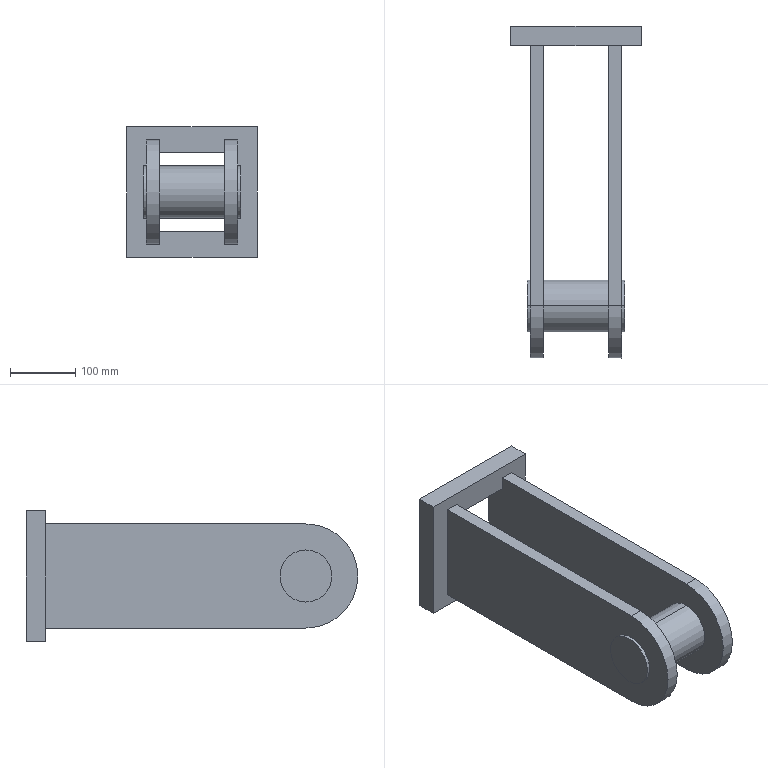Component | SolidWorks | LiftingAndOperatingMechanism-1_20-1 | 1 solid | 26 faces | box 200 x 510 x 200 mm | volume 4355044 mm3 | plane 18 | cylinder 8 | commonest cylinder face diameters 80 x6 160 x2
build123d program:
from build123d import *

# Parameters (mm, degrees)
SKETCH1_W           = 200
SKETCH1_H           = 200
BOSS_EXTRUDE1_DEPTH = 30
BOSS_EXTRUDE2_START = 50
BOSS_EXTRUDE2_DEPTH = 20
SKETCH4_R           = 40
BOSS_EXTRUDE3_DEPTH = 75
SKETCH5_W           = 120
SKETCH5_H           = 100
CUT_EXTRUDE2_DEPTH  = 501.4


with BuildPart() as part:
    # Sketch1 → Boss-Extrude1 (new body)
    with BuildSketch(Plane(origin=(0, 0, 0), x_dir=(1, 0, 0), z_dir=(0, 1, 0))):
        Rectangle(SKETCH1_W, SKETCH1_H)
    extrude(amount=BOSS_EXTRUDE1_DEPTH)

    # Sketch2 → Boss-Extrude2 (add)
    with BuildSketch(Plane.XY.offset(BOSS_EXTRUDE2_START)):
        with BuildLine():
            Line((-80, 430), (-80, 30))
            Line((-80, 30), (80, 30))
            Line((80, 30), (80, 430))
            ThreePointArc((80, 430), (0, 510), (-80, 430))
        make_face()
    boss_extrude2 = extrude(amount=BOSS_EXTRUDE2_DEPTH)

    # Mirror1: Boss-Extrude2 across plane
    add(boss_extrude2.mirror(Plane.XY))

    # Sketch4 → Boss-Extrude3 (add, symmetric)
    with BuildSketch(Plane.XY):
        with Locations(Location((0, 430, 0), (0, 0, 180))):
            Circle(SKETCH4_R)
    extrude(amount=BOSS_EXTRUDE3_DEPTH, both=True)

    # Sketch5 → Cut-Extrude2 (cut, through all)
    with BuildSketch(Plane(origin=(0, 30, 0), x_dir=(1, 0, 0), z_dir=(0, 1, 0))):
        Rectangle(SKETCH5_W, SKETCH5_H)
    extrude(amount=-CUT_EXTRUDE2_DEPTH, mode=Mode.SUBTRACT)


solid = part.part

# Placed as in the assembly
solid = solid.moved(Location((-1438.963, 12438.918, 6252.153), (180, 90, 0)))
STEP:
#1=COLOUR_RGB('',0.7922,0.8196,0.9333);
#2=FILL_AREA_STYLE_COLOUR('',#1);
#3=FILL_AREA_STYLE('',(#2));
#4=SURFACE_STYLE_FILL_AREA(#3);
#5=SURFACE_SIDE_STYLE('',(#4));
#6=SURFACE_STYLE_USAGE(.BOTH.,#5);
#7=PRESENTATION_STYLE_ASSIGNMENT((#6));
#8=CARTESIAN_POINT('',(-59.605,472.792,244.573));
#9=VERTEX_POINT('',#8);
#10=CARTESIAN_POINT('',(-59.605,472.792,247.723));
#11=VERTEX_POINT('',#10);
#12=CARTESIAN_POINT('',(-59.605,472.792,246.148));
#13=DIRECTION('',(-1.,-0.,0.0000002));
#14=DIRECTION('',(-0.0000002,0.,-1.));
#15=AXIS2_PLACEMENT_3D('',#12,#13,#14);
#16=CIRCLE('',#15,1.575);
#17=EDGE_CURVE('',#9,#11,#16,.T.);
#18=ORIENTED_EDGE('',*,*,#17,.F.);
#19=CARTESIAN_POINT('',(-59.408,472.792,244.573));
#20=VERTEX_POINT('',#19);
#21=CARTESIAN_POINT('',(-59.605,472.792,244.573));
#22=DIRECTION('',(1.,0.,-0.0000002));
#23=VECTOR('',#22,39.37);
#24=LINE('',#21,#23);
#25=EDGE_CURVE('',#9,#20,#24,.T.);
#26=ORIENTED_EDGE('',*,*,#25,.T.);
#27=CARTESIAN_POINT('',(-59.408,472.792,247.723));
#28=VERTEX_POINT('',#27);
#29=CARTESIAN_POINT('',(-59.408,472.792,246.148));
#30=DIRECTION('',(1.,0.,-0.0000002));
#31=DIRECTION('',(-0.0000002,0.,-1.));
#32=AXIS2_PLACEMENT_3D('',#29,#30,#31);
#33=CIRCLE('',#32,1.575);
#34=EDGE_CURVE('',#28,#20,#33,.T.);
#35=ORIENTED_EDGE('',*,*,#34,.F.);
#36=CARTESIAN_POINT('',(-59.605,472.792,247.723));
#37=DIRECTION('',(1.,0.,-0.0000002));
#38=VECTOR('',#37,39.37);
#39=LINE('',#36,#38);
#40=EDGE_CURVE('',#11,#28,#39,.T.);
#41=ORIENTED_EDGE('',*,*,#40,.F.);
#42=EDGE_LOOP('',(#18,#26,#35,#41));
#43=FACE_OUTER_BOUND('',#42,.T.);
#44=CARTESIAN_POINT('',(-59.605,472.792,246.148));
#45=DIRECTION('',(1.,0.,-0.0000002));
#46=DIRECTION('',(0.0000002,0.,1.));
#47=AXIS2_PLACEMENT_3D('',#44,#45,#46);
#48=CYLINDRICAL_SURFACE('',#47,1.575);
#49=ADVANCED_FACE('',(#43),#48,.T.);
#50=CARTESIAN_POINT('',(-53.896,472.792,244.573));
#51=VERTEX_POINT('',#50);
#52=CARTESIAN_POINT('',(-53.896,472.792,247.723));
#53=VERTEX_POINT('',#52);
#54=CARTESIAN_POINT('',(-53.896,472.792,246.148));
#55=DIRECTION('',(-1.,-0.,0.0000002));
#56=DIRECTION('',(0.0000002,0.,1.));
#57=AXIS2_PLACEMENT_3D('',#54,#55,#56);
#58=CIRCLE('',#57,1.575);
#59=EDGE_CURVE('',#51,#53,#58,.T.);
#60=ORIENTED_EDGE('',*,*,#59,.F.);
#61=CARTESIAN_POINT('',(-53.699,472.792,244.573));
#62=VERTEX_POINT('',#61);
#63=CARTESIAN_POINT('',(-59.605,472.792,244.573));
#64=DIRECTION('',(1.,0.,-0.0000002));
#65=VECTOR('',#64,39.37);
#66=LINE('',#63,#65);
#67=EDGE_CURVE('',#51,#62,#66,.T.);
#68=ORIENTED_EDGE('',*,*,#67,.T.);
#69=CARTESIAN_POINT('',(-53.699,472.792,247.723));
#70=VERTEX_POINT('',#69);
#71=CARTESIAN_POINT('',(-53.699,472.792,246.148));
#72=DIRECTION('',(-1.,-0.,0.0000002));
#73=DIRECTION('',(-0.0000002,0.,-1.));
#74=AXIS2_PLACEMENT_3D('',#71,#72,#73);
#75=CIRCLE('',#74,1.575);
#76=EDGE_CURVE('',#62,#70,#75,.T.);
#77=ORIENTED_EDGE('',*,*,#76,.T.);
#78=CARTESIAN_POINT('',(-59.605,472.792,247.723));
#79=DIRECTION('',(1.,0.,-0.0000002));
#80=VECTOR('',#79,39.37);
#81=LINE('',#78,#80);
#82=EDGE_CURVE('',#53,#70,#81,.T.);
#83=ORIENTED_EDGE('',*,*,#82,.F.);
#84=EDGE_LOOP('',(#60,#68,#77,#83));
#85=FACE_OUTER_BOUND('',#84,.T.);
#86=CARTESIAN_POINT('',(-59.605,472.792,246.148));
#87=DIRECTION('',(1.,0.,-0.0000002));
#88=DIRECTION('',(0.0000002,0.,1.));
#89=AXIS2_PLACEMENT_3D('',#86,#87,#88);
#90=CYLINDRICAL_SURFACE('',#89,1.575);
#91=ADVANCED_FACE('',(#85),#90,.T.);
#92=CARTESIAN_POINT('',(-58.621,472.792,247.723));
#93=VERTEX_POINT('',#92);
#94=CARTESIAN_POINT('',(-58.621,472.792,244.573));
#95=VERTEX_POINT('',#94);
#96=CARTESIAN_POINT('',(-58.621,472.792,246.148));
#97=DIRECTION('',(1.,0.,-0.0000002));
#98=DIRECTION('',(-0.0000002,0.,-1.));
#99=AXIS2_PLACEMENT_3D('',#96,#97,#98);
#100=CIRCLE('',#99,1.575);
#101=EDGE_CURVE('',#93,#95,#100,.T.);
#102=ORIENTED_EDGE('',*,*,#101,.T.);
#103=CARTESIAN_POINT('',(-54.684,472.792,244.573));
#104=VERTEX_POINT('',#103);
#105=CARTESIAN_POINT('',(-59.605,472.792,244.573));
#106=DIRECTION('',(1.,0.,-0.0000002));
#107=VECTOR('',#106,39.37);
#108=LINE('',#105,#107);
#109=EDGE_CURVE('',#95,#104,#108,.T.);
#110=ORIENTED_EDGE('',*,*,#109,.T.);
#111=CARTESIAN_POINT('',(-54.684,472.792,247.723));
#112=VERTEX_POINT('',#111);
#113=CARTESIAN_POINT('',(-54.684,472.792,246.148));
#114=DIRECTION('',(-1.,-0.,0.0000002));
#115=DIRECTION('',(0.0000002,0.,1.));
#116=AXIS2_PLACEMENT_3D('',#113,#114,#115);
#117=CIRCLE('',#116,1.575);
#118=EDGE_CURVE('',#104,#112,#117,.T.);
#119=ORIENTED_EDGE('',*,*,#118,.T.);
#120=CARTESIAN_POINT('',(-59.605,472.792,247.723));
#121=DIRECTION('',(1.,0.,-0.0000002));
#122=VECTOR('',#121,39.37);
#123=LINE('',#120,#122);
#124=EDGE_CURVE('',#93,#112,#123,.T.);
#125=ORIENTED_EDGE('',*,*,#124,.F.);
#126=EDGE_LOOP('',(#102,#110,#119,#125));
#127=FACE_OUTER_BOUND('',#126,.T.);
#128=CARTESIAN_POINT('',(-59.605,472.792,246.148));
#129=DIRECTION('',(1.,0.,-0.0000002));
#130=DIRECTION('',(0.0000002,0.,1.));
#131=AXIS2_PLACEMENT_3D('',#128,#129,#130);
#132=CYLINDRICAL_SURFACE('',#131,1.575);
#133=ADVANCED_FACE('',(#127),#132,.T.);
#134=CARTESIAN_POINT('',(-60.589,489.721,242.211));
#135=VERTEX_POINT('',#134);
#136=CARTESIAN_POINT('',(-52.715,489.721,242.211));
#137=VERTEX_POINT('',#136);
#138=CARTESIAN_POINT('',(-52.715,489.721,242.211));
#139=DIRECTION('',(1.,0.,-0.0000002));
#140=VECTOR('',#139,39.37);
#141=LINE('',#138,#140);
#142=EDGE_CURVE('',#135,#137,#141,.T.);
#143=ORIENTED_EDGE('',*,*,#142,.T.);
#144=CARTESIAN_POINT('',(-52.715,488.54,242.211));
#145=VERTEX_POINT('',#144);
#146=CARTESIAN_POINT('',(-52.715,488.54,242.211));
#147=DIRECTION('',(-0.,1.,0.));
#148=VECTOR('',#147,39.37);
#149=LINE('',#146,#148);
#150=EDGE_CURVE('',#145,#137,#149,.T.);
#151=ORIENTED_EDGE('',*,*,#150,.F.);
#152=CARTESIAN_POINT('',(-60.589,488.54,242.211));
#153=VERTEX_POINT('',#152);
#154=CARTESIAN_POINT('',(-52.715,488.54,242.211));
#155=DIRECTION('',(1.,0.,-0.0000002));
#156=VECTOR('',#155,39.37);
#157=LINE('',#154,#156);
#158=EDGE_CURVE('',#153,#145,#157,.T.);
#159=ORIENTED_EDGE('',*,*,#158,.F.);
#160=CARTESIAN_POINT('',(-60.589,488.54,242.211));
#161=DIRECTION('',(-0.,1.,0.));
#162=VECTOR('',#161,39.37);
#163=LINE('',#160,#162);
#164=EDGE_CURVE('',#153,#135,#163,.T.);
#165=ORIENTED_EDGE('',*,*,#164,.T.);
#166=EDGE_LOOP('',(#143,#151,#159,#165));
#167=FACE_OUTER_BOUND('',#166,.T.);
#168=CARTESIAN_POINT('',(-52.715,488.54,242.211));
#169=DIRECTION('',(0.0000002,-0.,1.));
#170=DIRECTION('',(-1.,-0.,0.0000002));
#171=AXIS2_PLACEMENT_3D('',#168,#169,#170);
#172=PLANE('',#171);
#173=ADVANCED_FACE('',(#167),#172,.F.);
#174=CARTESIAN_POINT('',(-52.715,489.721,250.085));
#175=VERTEX_POINT('',#174);
#176=CARTESIAN_POINT('',(-52.715,489.721,250.085));
#177=DIRECTION('',(0.0000002,-0.,1.));
#178=VECTOR('',#177,39.37);
#179=LINE('',#176,#178);
#180=EDGE_CURVE('',#137,#175,#179,.T.);
#181=ORIENTED_EDGE('',*,*,#180,.T.);
#182=CARTESIAN_POINT('',(-52.715,488.54,250.085));
#183=VERTEX_POINT('',#182);
#184=CARTESIAN_POINT('',(-52.715,488.54,250.085));
#185=DIRECTION('',(-0.,1.,0.));
#186=VECTOR('',#185,39.37);
#187=LINE('',#184,#186);
#188=EDGE_CURVE('',#183,#175,#187,.T.);
#189=ORIENTED_EDGE('',*,*,#188,.F.);
#190=CARTESIAN_POINT('',(-52.715,488.54,250.085));
#191=DIRECTION('',(0.0000002,-0.,1.));
#192=VECTOR('',#191,39.37);
#193=LINE('',#190,#192);
#194=EDGE_CURVE('',#145,#183,#193,.T.);
#195=ORIENTED_EDGE('',*,*,#194,.F.);
#196=ORIENTED_EDGE('',*,*,#150,.T.);
#197=EDGE_LOOP('',(#181,#189,#195,#196));
#198=FACE_OUTER_BOUND('',#197,.T.);
#199=CARTESIAN_POINT('',(-52.715,488.54,250.085));
#200=DIRECTION('',(-1.,-0.,0.0000002));
#201=DIRECTION('',(-0.0000002,0.,-1.));
#202=AXIS2_PLACEMENT_3D('',#199,#200,#201);
#203=PLANE('',#202);
#204=ADVANCED_FACE('',(#198),#203,.F.);
#205=CARTESIAN_POINT('',(-60.589,489.721,250.085));
#206=VERTEX_POINT('',#205);
#207=CARTESIAN_POINT('',(-52.715,489.721,250.085));
#208=DIRECTION('',(-1.,-0.,0.0000002));
#209=VECTOR('',#208,39.37);
#210=LINE('',#207,#209);
#211=EDGE_CURVE('',#175,#206,#210,.T.);
#212=ORIENTED_EDGE('',*,*,#211,.T.);
#213=CARTESIAN_POINT('',(-60.589,488.54,250.085));
#214=VERTEX_POINT('',#213);
#215=CARTESIAN_POINT('',(-60.589,488.54,250.085));
#216=DIRECTION('',(-0.,1.,0.));
#217=VECTOR('',#216,39.37);
#218=LINE('',#215,#217);
#219=EDGE_CURVE('',#214,#206,#218,.T.);
#220=ORIENTED_EDGE('',*,*,#219,.F.);
#221=CARTESIAN_POINT('',(-52.715,488.54,250.085));
#222=DIRECTION('',(-1.,-0.,0.0000002));
#223=VECTOR('',#222,39.37);
#224=LINE('',#221,#223);
#225=EDGE_CURVE('',#183,#214,#224,.T.);
#226=ORIENTED_EDGE('',*,*,#225,.F.);
#227=ORIENTED_EDGE('',*,*,#188,.T.);
#228=EDGE_LOOP('',(#212,#220,#226,#227));
#229=FACE_OUTER_BOUND('',#228,.T.);
#230=CARTESIAN_POINT('',(-52.715,488.54,250.085));
#231=DIRECTION('',(-0.0000002,0.,-1.));
#232=DIRECTION('',(1.,0.,-0.0000002));
#233=AXIS2_PLACEMENT_3D('',#230,#231,#232);
#234=PLANE('',#233);
#235=ADVANCED_FACE('',(#229),#234,.F.);
#236=CARTESIAN_POINT('',(-60.589,489.721,250.085));
#237=DIRECTION('',(-0.0000002,0.,-1.));
#238=VECTOR('',#237,39.37);
#239=LINE('',#236,#238);
#240=EDGE_CURVE('',#206,#135,#239,.T.);
#241=ORIENTED_EDGE('',*,*,#240,.T.);
#242=ORIENTED_EDGE('',*,*,#164,.F.);
#243=CARTESIAN_POINT('',(-60.589,488.54,250.085));
#244=DIRECTION('',(-0.0000002,0.,-1.));
#245=VECTOR('',#244,39.37);
#246=LINE('',#243,#245);
#247=EDGE_CURVE('',#214,#153,#246,.T.);
#248=ORIENTED_EDGE('',*,*,#247,.F.);
#249=ORIENTED_EDGE('',*,*,#219,.T.);
#250=EDGE_LOOP('',(#241,#242,#248,#249));
#251=FACE_OUTER_BOUND('',#250,.T.);
#252=CARTESIAN_POINT('',(-60.589,488.54,250.085));
#253=DIRECTION('',(1.,0.,-0.0000002));
#254=DIRECTION('',(0.0000002,-0.,1.));
#255=AXIS2_PLACEMENT_3D('',#252,#253,#254);
#256=PLANE('',#255);
#257=ADVANCED_FACE('',(#251),#256,.F.);
#258=CARTESIAN_POINT('',(-58.621,488.54,243.786));
#259=VERTEX_POINT('',#258);
#260=CARTESIAN_POINT('',(-54.684,488.54,243.786));
#261=VERTEX_POINT('',#260);
#262=CARTESIAN_POINT('',(-54.684,488.54,243.786));
#263=DIRECTION('',(1.,0.,-0.0000002));
#264=VECTOR('',#263,39.37);
#265=LINE('',#262,#264);
#266=EDGE_CURVE('',#259,#261,#265,.T.);
#267=ORIENTED_EDGE('',*,*,#266,.F.);
#268=CARTESIAN_POINT('',(-58.621,488.54,242.998));
#269=VERTEX_POINT('',#268);
#270=CARTESIAN_POINT('',(-58.621,488.54,246.148));
#271=DIRECTION('',(-0.0000002,-0.,-1.));
#272=VECTOR('',#271,39.37);
#273=LINE('',#270,#272);
#274=EDGE_CURVE('',#259,#269,#273,.T.);
#275=ORIENTED_EDGE('',*,*,#274,.T.);
#276=CARTESIAN_POINT('',(-59.408,488.54,242.998));
#277=VERTEX_POINT('',#276);
#278=CARTESIAN_POINT('',(-59.408,488.54,242.998));
#279=DIRECTION('',(1.,0.,-0.0000002));
#280=VECTOR('',#279,39.37);
#281=LINE('',#278,#280);
#282=EDGE_CURVE('',#277,#269,#281,.T.);
#283=ORIENTED_EDGE('',*,*,#282,.F.);
#284=CARTESIAN_POINT('',(-59.408,488.54,249.297));
#285=VERTEX_POINT('',#284);
#286=CARTESIAN_POINT('',(-59.408,488.54,246.148));
#287=DIRECTION('',(-0.0000002,-0.,-1.));
#288=VECTOR('',#287,39.37);
#289=LINE('',#286,#288);
#290=EDGE_CURVE('',#285,#277,#289,.T.);
#291=ORIENTED_EDGE('',*,*,#290,.F.);
#292=CARTESIAN_POINT('',(-58.621,488.54,249.297));
#293=VERTEX_POINT('',#292);
#294=CARTESIAN_POINT('',(-59.408,488.54,249.297));
#295=DIRECTION('',(1.,0.,-0.0000002));
#296=VECTOR('',#295,39.37);
#297=LINE('',#294,#296);
#298=EDGE_CURVE('',#285,#293,#297,.T.);
#299=ORIENTED_EDGE('',*,*,#298,.T.);
#300=CARTESIAN_POINT('',(-58.621,488.54,248.51));
#301=VERTEX_POINT('',#300);
#302=CARTESIAN_POINT('',(-58.621,488.54,246.148));
#303=DIRECTION('',(-0.0000002,-0.,-1.));
#304=VECTOR('',#303,39.37);
#305=LINE('',#302,#304);
#306=EDGE_CURVE('',#293,#301,#305,.T.);
#307=ORIENTED_EDGE('',*,*,#306,.T.);
#308=CARTESIAN_POINT('',(-54.684,488.54,248.51));
#309=VERTEX_POINT('',#308);
#310=CARTESIAN_POINT('',(-54.684,488.54,248.51));
#311=DIRECTION('',(-1.,-0.,0.0000002));
#312=VECTOR('',#311,39.37);
#313=LINE('',#310,#312);
#314=EDGE_CURVE('',#309,#301,#313,.T.);
#315=ORIENTED_EDGE('',*,*,#314,.F.);
#316=CARTESIAN_POINT('',(-54.684,488.54,249.297));
#317=VERTEX_POINT('',#316);
#318=CARTESIAN_POINT('',(-54.684,488.54,246.148));
#319=DIRECTION('',(-0.0000002,-0.,-1.));
#320=VECTOR('',#319,39.37);
#321=LINE('',#318,#320);
#322=EDGE_CURVE('',#317,#309,#321,.T.);
#323=ORIENTED_EDGE('',*,*,#322,.F.);
#324=CARTESIAN_POINT('',(-53.896,488.54,249.297));
#325=VERTEX_POINT('',#324);
#326=CARTESIAN_POINT('',(-53.896,488.54,249.297));
#327=DIRECTION('',(-1.,-0.,0.0000002));
#328=VECTOR('',#327,39.37);
#329=LINE('',#326,#328);
#330=EDGE_CURVE('',#325,#317,#329,.T.);
#331=ORIENTED_EDGE('',*,*,#330,.F.);
#332=CARTESIAN_POINT('',(-53.896,488.54,242.998));
#333=VERTEX_POINT('',#332);
#334=CARTESIAN_POINT('',(-53.896,488.54,246.148));
#335=DIRECTION('',(-0.0000002,-0.,-1.));
#336=VECTOR('',#335,39.37);
#337=LINE('',#334,#336);
#338=EDGE_CURVE('',#325,#333,#337,.T.);
#339=ORIENTED_EDGE('',*,*,#338,.T.);
#340=CARTESIAN_POINT('',(-54.684,488.54,242.998));
#341=VERTEX_POINT('',#340);
#342=CARTESIAN_POINT('',(-53.896,488.54,242.998));
#343=DIRECTION('',(-1.,-0.,0.0000002));
#344=VECTOR('',#343,39.37);
#345=LINE('',#342,#344);
#346=EDGE_CURVE('',#333,#341,#345,.T.);
#347=ORIENTED_EDGE('',*,*,#346,.T.);
#348=CARTESIAN_POINT('',(-54.684,488.54,246.148));
#349=DIRECTION('',(-0.0000002,-0.,-1.));
#350=VECTOR('',#349,39.37);
#351=LINE('',#348,#350);
#352=EDGE_CURVE('',#261,#341,#351,.T.);
#353=ORIENTED_EDGE('',*,*,#352,.F.);
#354=EDGE_LOOP('',(#267,#275,#283,#291,#299,#307,#315,#323,#331,#339,#347,#353));
#355=FACE_BOUND('',#354,.T.);
#356=ORIENTED_EDGE('',*,*,#158,.T.);
#357=ORIENTED_EDGE('',*,*,#194,.T.);
#358=ORIENTED_EDGE('',*,*,#225,.T.);
#359=ORIENTED_EDGE('',*,*,#247,.T.);
#360=EDGE_LOOP('',(#356,#357,#358,#359));
#361=FACE_OUTER_BOUND('',#360,.T.);
#362=CARTESIAN_POINT('',(-56.652,488.54,246.148));
#363=DIRECTION('',(0.,-1.,-0.));
#364=DIRECTION('',(-1.,-0.,0.0000002));
#365=AXIS2_PLACEMENT_3D('',#362,#363,#364);
#366=PLANE('',#365);
#367=ADVANCED_FACE('',(#355,#361),#366,.T.);
#368=CARTESIAN_POINT('',(-58.621,489.721,248.51));
#369=VERTEX_POINT('',#368);
#370=CARTESIAN_POINT('',(-58.621,489.721,243.786));
#371=VERTEX_POINT('',#370);
#372=CARTESIAN_POINT('',(-58.621,489.721,248.51));
#373=DIRECTION('',(-0.0000002,0.,-1.));
#374=VECTOR('',#373,39.37);
#375=LINE('',#372,#374);
#376=EDGE_CURVE('',#369,#371,#375,.T.);
#377=ORIENTED_EDGE('',*,*,#376,.T.);
#378=CARTESIAN_POINT('',(-54.684,489.721,243.786));
#379=VERTEX_POINT('',#378);
#380=CARTESIAN_POINT('',(-54.684,489.721,243.786));
#381=DIRECTION('',(1.,0.,-0.0000002));
#382=VECTOR('',#381,39.37);
#383=LINE('',#380,#382);
#384=EDGE_CURVE('',#371,#379,#383,.T.);
#385=ORIENTED_EDGE('',*,*,#384,.T.);
#386=CARTESIAN_POINT('',(-54.684,489.721,248.51));
#387=VERTEX_POINT('',#386);
#388=CARTESIAN_POINT('',(-54.684,489.721,248.51));
#389=DIRECTION('',(0.0000002,-0.,1.));
#390=VECTOR('',#389,39.37);
#391=LINE('',#388,#390);
#392=EDGE_CURVE('',#379,#387,#391,.T.);
#393=ORIENTED_EDGE('',*,*,#392,.T.);
#394=CARTESIAN_POINT('',(-54.684,489.721,248.51));
#395=DIRECTION('',(-1.,-0.,0.0000002));
#396=VECTOR('',#395,39.37);
#397=LINE('',#394,#396);
#398=EDGE_CURVE('',#387,#369,#397,.T.);
#399=ORIENTED_EDGE('',*,*,#398,.T.);
#400=EDGE_LOOP('',(#377,#385,#393,#399));
#401=FACE_BOUND('',#400,.T.);
#402=ORIENTED_EDGE('',*,*,#142,.F.);
#403=ORIENTED_EDGE('',*,*,#240,.F.);
#404=ORIENTED_EDGE('',*,*,#211,.F.);
#405=ORIENTED_EDGE('',*,*,#180,.F.);
#406=EDGE_LOOP('',(#402,#403,#404,#405));
#407=FACE_OUTER_BOUND('',#406,.T.);
#408=CARTESIAN_POINT('',(-56.652,489.721,246.148));
#409=DIRECTION('',(0.,-1.,-0.));
#410=DIRECTION('',(-1.,-0.,0.0000002));
#411=AXIS2_PLACEMENT_3D('',#408,#409,#410);
#412=PLANE('',#411);
#413=ADVANCED_FACE('',(#401,#407),#412,.F.);
#414=CARTESIAN_POINT('',(-58.621,472.792,242.998));
#415=VERTEX_POINT('',#414);
#416=CARTESIAN_POINT('',(-58.621,489.721,242.998));
#417=DIRECTION('',(0.,-1.,-0.));
#418=VECTOR('',#417,39.37);
#419=LINE('',#416,#418);
#420=EDGE_CURVE('',#269,#415,#419,.T.);
#421=ORIENTED_EDGE('',*,*,#420,.T.);
#422=CARTESIAN_POINT('',(-59.408,472.792,242.998));
#423=VERTEX_POINT('',#422);
#424=CARTESIAN_POINT('',(-59.408,472.792,242.998));
#425=DIRECTION('',(1.,0.,-0.0000002));
#426=VECTOR('',#425,39.37);
#427=LINE('',#424,#426);
#428=EDGE_CURVE('',#423,#415,#427,.T.);
#429=ORIENTED_EDGE('',*,*,#428,.F.);
#430=CARTESIAN_POINT('',(-59.408,489.721,242.998));
#431=DIRECTION('',(0.,-1.,-0.));
#432=VECTOR('',#431,39.37);
#433=LINE('',#430,#432);
#434=EDGE_CURVE('',#277,#423,#433,.T.);
#435=ORIENTED_EDGE('',*,*,#434,.F.);
#436=ORIENTED_EDGE('',*,*,#282,.T.);
#437=EDGE_LOOP('',(#421,#429,#435,#436));
#438=FACE_OUTER_BOUND('',#437,.T.);
#439=CARTESIAN_POINT('',(-59.408,489.721,242.998));
#440=DIRECTION('',(0.0000002,-0.,1.));
#441=DIRECTION('',(-1.,-0.,0.0000002));
#442=AXIS2_PLACEMENT_3D('',#439,#440,#441);
#443=PLANE('',#442);
#444=ADVANCED_FACE('',(#438),#443,.F.);
#445=CARTESIAN_POINT('',(-58.621,472.792,249.297));
#446=VERTEX_POINT('',#445);
#447=CARTESIAN_POINT('',(-58.621,472.792,246.148));
#448=DIRECTION('',(-1.,-0.,0.0000002));
#449=DIRECTION('',(-0.0000002,0.,-1.));
#450=AXIS2_PLACEMENT_3D('',#447,#448,#449);
#451=CIRCLE('',#450,3.15);
#452=EDGE_CURVE('',#415,#446,#451,.T.);
#453=ORIENTED_EDGE('',*,*,#452,.T.);
#454=CARTESIAN_POINT('',(-59.408,472.792,249.297));
#455=VERTEX_POINT('',#454);
#456=CARTESIAN_POINT('',(-59.408,472.792,249.297));
#457=DIRECTION('',(1.,0.,-0.0000002));
#458=VECTOR('',#457,39.37);
#459=LINE('',#456,#458);
#460=EDGE_CURVE('',#455,#446,#459,.T.);
#461=ORIENTED_EDGE('',*,*,#460,.F.);
#462=CARTESIAN_POINT('',(-59.408,472.792,246.148));
#463=DIRECTION('',(-1.,-0.,0.0000002));
#464=DIRECTION('',(-0.0000002,0.,-1.));
#465=AXIS2_PLACEMENT_3D('',#462,#463,#464);
#466=CIRCLE('',#465,3.15);
#467=EDGE_CURVE('',#423,#455,#466,.T.);
#468=ORIENTED_EDGE('',*,*,#467,.F.);
#469=ORIENTED_EDGE('',*,*,#428,.T.);
#470=EDGE_LOOP('',(#453,#461,#468,#469));
#471=FACE_OUTER_BOUND('',#470,.T.);
#472=CARTESIAN_POINT('',(-59.408,472.792,246.148));
#473=DIRECTION('',(1.,0.,-0.0000002));
#474=DIRECTION('',(0.0000002,0.,1.));
#475=AXIS2_PLACEMENT_3D('',#472,#473,#474);
#476=CYLINDRICAL_SURFACE('',#475,3.15);
#477=ADVANCED_FACE('',(#471),#476,.T.);
#478=CARTESIAN_POINT('',(-58.621,489.721,249.297));
#479=DIRECTION('',(0.,-1.,-0.));
#480=VECTOR('',#479,39.37);
#481=LINE('',#478,#480);
#482=EDGE_CURVE('',#293,#446,#481,.T.);
#483=ORIENTED_EDGE('',*,*,#482,.F.);
#484=ORIENTED_EDGE('',*,*,#298,.F.);
#485=CARTESIAN_POINT('',(-59.408,489.721,249.297));
#486=DIRECTION('',(0.,-1.,-0.));
#487=VECTOR('',#486,39.37);
#488=LINE('',#485,#487);
#489=EDGE_CURVE('',#285,#455,#488,.T.);
#490=ORIENTED_EDGE('',*,*,#489,.T.);
#491=ORIENTED_EDGE('',*,*,#460,.T.);
#492=EDGE_LOOP('',(#483,#484,#490,#491));
#493=FACE_OUTER_BOUND('',#492,.T.);
#494=CARTESIAN_POINT('',(-59.408,489.721,249.297));
#495=DIRECTION('',(0.0000002,-0.,1.));
#496=DIRECTION('',(-1.,-0.,0.0000002));
#497=AXIS2_PLACEMENT_3D('',#494,#495,#496);
#498=PLANE('',#497);
#499=ADVANCED_FACE('',(#493),#498,.T.);
#500=ORIENTED_EDGE('',*,*,#34,.T.);
#501=CARTESIAN_POINT('',(-59.408,472.792,246.148));
#502=DIRECTION('',(1.,0.,-0.0000002));
#503=DIRECTION('',(-0.0000002,0.,-1.));
#504=AXIS2_PLACEMENT_3D('',#501,#502,#503);
#505=CIRCLE('',#504,1.575);
#506=EDGE_CURVE('',#20,#28,#505,.T.);
#507=ORIENTED_EDGE('',*,*,#506,.T.);
#508=EDGE_LOOP('',(#500,#507));
#509=FACE_BOUND('',#508,.T.);
#510=ORIENTED_EDGE('',*,*,#434,.T.);
#511=ORIENTED_EDGE('',*,*,#467,.T.);
#512=ORIENTED_EDGE('',*,*,#489,.F.);
#513=ORIENTED_EDGE('',*,*,#290,.T.);
#514=EDGE_LOOP('',(#510,#511,#512,#513));
#515=FACE_OUTER_BOUND('',#514,.T.);
#516=CARTESIAN_POINT('',(-59.408,489.721,246.148));
#517=DIRECTION('',(-1.,-0.,0.0000002));
#518=DIRECTION('',(-0.0000002,0.,-1.));
#519=AXIS2_PLACEMENT_3D('',#516,#517,#518);
#520=PLANE('',#519);
#521=ADVANCED_FACE('',(#509,#515),#520,.T.);
#522=ORIENTED_EDGE('',*,*,#101,.F.);
#523=CARTESIAN_POINT('',(-58.621,472.792,246.148));
#524=DIRECTION('',(1.,0.,-0.0000002));
#525=DIRECTION('',(-0.0000002,0.,-1.));
#526=AXIS2_PLACEMENT_3D('',#523,#524,#525);
#527=CIRCLE('',#526,1.575);
#528=EDGE_CURVE('',#95,#93,#527,.T.);
#529=ORIENTED_EDGE('',*,*,#528,.F.);
#530=EDGE_LOOP('',(#522,#529));
#531=FACE_BOUND('',#530,.T.);
#532=ORIENTED_EDGE('',*,*,#420,.F.);
#533=ORIENTED_EDGE('',*,*,#274,.F.);
#534=CARTESIAN_POINT('',(-58.621,489.721,243.786));
#535=DIRECTION('',(0.,-1.,-0.));
#536=VECTOR('',#535,39.37);
#537=LINE('',#534,#536);
#538=EDGE_CURVE('',#371,#259,#537,.T.);
#539=ORIENTED_EDGE('',*,*,#538,.F.);
#540=ORIENTED_EDGE('',*,*,#376,.F.);
#541=CARTESIAN_POINT('',(-58.621,489.721,248.51));
#542=DIRECTION('',(0.,-1.,-0.));
#543=VECTOR('',#542,39.37);
#544=LINE('',#541,#543);
#545=EDGE_CURVE('',#369,#301,#544,.T.);
#546=ORIENTED_EDGE('',*,*,#545,.T.);
#547=ORIENTED_EDGE('',*,*,#306,.F.);
#548=ORIENTED_EDGE('',*,*,#482,.T.);
#549=ORIENTED_EDGE('',*,*,#452,.F.);
#550=EDGE_LOOP('',(#532,#533,#539,#540,#546,#547,#548,#549));
#551=FACE_OUTER_BOUND('',#550,.T.);
#552=CARTESIAN_POINT('',(-58.621,489.721,246.148));
#553=DIRECTION('',(-1.,-0.,0.0000002));
#554=DIRECTION('',(-0.0000002,0.,-1.));
#555=AXIS2_PLACEMENT_3D('',#552,#553,#554);
#556=PLANE('',#555);
#557=ADVANCED_FACE('',(#531,#551),#556,.F.);
#558=CARTESIAN_POINT('',(-54.684,472.792,242.998));
#559=VERTEX_POINT('',#558);
#560=CARTESIAN_POINT('',(-54.684,489.721,242.998));
#561=DIRECTION('',(0.,-1.,-0.));
#562=VECTOR('',#561,39.37);
#563=LINE('',#560,#562);
#564=EDGE_CURVE('',#341,#559,#563,.T.);
#565=ORIENTED_EDGE('',*,*,#564,.F.);
#566=ORIENTED_EDGE('',*,*,#346,.F.);
#567=CARTESIAN_POINT('',(-53.896,472.792,242.998));
#568=VERTEX_POINT('',#567);
#569=CARTESIAN_POINT('',(-53.896,489.721,242.998));
#570=DIRECTION('',(0.,-1.,-0.));
#571=VECTOR('',#570,39.37);
#572=LINE('',#569,#571);
#573=EDGE_CURVE('',#333,#568,#572,.T.);
#574=ORIENTED_EDGE('',*,*,#573,.T.);
#575=CARTESIAN_POINT('',(-53.896,472.792,242.998));
#576=DIRECTION('',(-1.,-0.,0.0000002));
#577=VECTOR('',#576,39.37);
#578=LINE('',#575,#577);
#579=EDGE_CURVE('',#568,#559,#578,.T.);
#580=ORIENTED_EDGE('',*,*,#579,.T.);
#581=EDGE_LOOP('',(#565,#566,#574,#580));
#582=FACE_OUTER_BOUND('',#581,.T.);
#583=CARTESIAN_POINT('',(-53.896,489.721,242.998));
#584=DIRECTION('',(-0.0000002,0.,-1.));
#585=DIRECTION('',(1.,0.,-0.0000002));
#586=AXIS2_PLACEMENT_3D('',#583,#584,#585);
#587=PLANE('',#586);
#588=ADVANCED_FACE('',(#582),#587,.T.);
#589=CARTESIAN_POINT('',(-54.684,472.792,249.297));
#590=VERTEX_POINT('',#589);
#591=CARTESIAN_POINT('',(-54.684,489.721,249.297));
#592=DIRECTION('',(0.,-1.,-0.));
#593=VECTOR('',#592,39.37);
#594=LINE('',#591,#593);
#595=EDGE_CURVE('',#317,#590,#594,.T.);
#596=ORIENTED_EDGE('',*,*,#595,.T.);
#597=CARTESIAN_POINT('',(-53.896,472.792,249.297));
#598=VERTEX_POINT('',#597);
#599=CARTESIAN_POINT('',(-53.896,472.792,249.297));
#600=DIRECTION('',(-1.,-0.,0.0000002));
#601=VECTOR('',#600,39.37);
#602=LINE('',#599,#601);
#603=EDGE_CURVE('',#598,#590,#602,.T.);
#604=ORIENTED_EDGE('',*,*,#603,.F.);
#605=CARTESIAN_POINT('',(-53.896,489.721,249.297));
#606=DIRECTION('',(0.,-1.,-0.));
#607=VECTOR('',#606,39.37);
#608=LINE('',#605,#607);
#609=EDGE_CURVE('',#325,#598,#608,.T.);
#610=ORIENTED_EDGE('',*,*,#609,.F.);
#611=ORIENTED_EDGE('',*,*,#330,.T.);
#612=EDGE_LOOP('',(#596,#604,#610,#611));
#613=FACE_OUTER_BOUND('',#612,.T.);
#614=CARTESIAN_POINT('',(-53.896,489.721,249.297));
#615=DIRECTION('',(-0.0000002,0.,-1.));
#616=DIRECTION('',(1.,0.,-0.0000002));
#617=AXIS2_PLACEMENT_3D('',#614,#615,#616);
#618=PLANE('',#617);
#619=ADVANCED_FACE('',(#613),#618,.F.);
#620=CARTESIAN_POINT('',(-54.684,472.792,246.148));
#621=DIRECTION('',(-1.,-0.,0.0000002));
#622=DIRECTION('',(-0.0000002,0.,-1.));
#623=AXIS2_PLACEMENT_3D('',#620,#621,#622);
#624=CIRCLE('',#623,3.15);
#625=EDGE_CURVE('',#559,#590,#624,.T.);
#626=ORIENTED_EDGE('',*,*,#625,.F.);
#627=ORIENTED_EDGE('',*,*,#579,.F.);
#628=CARTESIAN_POINT('',(-53.896,472.792,246.148));
#629=DIRECTION('',(-1.,-0.,0.0000002));
#630=DIRECTION('',(-0.0000002,0.,-1.));
#631=AXIS2_PLACEMENT_3D('',#628,#629,#630);
#632=CIRCLE('',#631,3.15);
#633=EDGE_CURVE('',#568,#598,#632,.T.);
#634=ORIENTED_EDGE('',*,*,#633,.T.);
#635=ORIENTED_EDGE('',*,*,#603,.T.);
#636=EDGE_LOOP('',(#626,#627,#634,#635));
#637=FACE_OUTER_BOUND('',#636,.T.);
#638=CARTESIAN_POINT('',(-53.896,472.792,246.148));
#639=DIRECTION('',(-1.,-0.,0.0000002));
#640=DIRECTION('',(-0.0000002,0.,-1.));
#641=AXIS2_PLACEMENT_3D('',#638,#639,#640);
#642=CYLINDRICAL_SURFACE('',#641,3.15);
#643=ADVANCED_FACE('',(#637),#642,.T.);
#644=CARTESIAN_POINT('',(-53.896,472.792,246.148));
#645=DIRECTION('',(-1.,-0.,0.0000002));
#646=DIRECTION('',(0.0000002,0.,1.));
#647=AXIS2_PLACEMENT_3D('',#644,#645,#646);
#648=CIRCLE('',#647,1.575);
#649=EDGE_CURVE('',#53,#51,#648,.T.);
#650=ORIENTED_EDGE('',*,*,#649,.T.);
#651=ORIENTED_EDGE('',*,*,#59,.T.);
#652=EDGE_LOOP('',(#650,#651));
#653=FACE_BOUND('',#652,.T.);
#654=ORIENTED_EDGE('',*,*,#573,.F.);
#655=ORIENTED_EDGE('',*,*,#338,.F.);
#656=ORIENTED_EDGE('',*,*,#609,.T.);
#657=ORIENTED_EDGE('',*,*,#633,.F.);
#658=EDGE_LOOP('',(#654,#655,#656,#657));
#659=FACE_OUTER_BOUND('',#658,.T.);
#660=CARTESIAN_POINT('',(-53.896,489.721,246.148));
#661=DIRECTION('',(1.,0.,-0.0000002));
#662=DIRECTION('',(-0.0000002,0.,-1.));
#663=AXIS2_PLACEMENT_3D('',#660,#661,#662);
#664=PLANE('',#663);
#665=ADVANCED_FACE('',(#653,#659),#664,.T.);
#666=CARTESIAN_POINT('',(-54.684,472.792,246.148));
#667=DIRECTION('',(-1.,-0.,0.0000002));
#668=DIRECTION('',(0.0000002,0.,1.));
#669=AXIS2_PLACEMENT_3D('',#666,#667,#668);
#670=CIRCLE('',#669,1.575);
#671=EDGE_CURVE('',#112,#104,#670,.T.);
#672=ORIENTED_EDGE('',*,*,#671,.F.);
#673=ORIENTED_EDGE('',*,*,#118,.F.);
#674=EDGE_LOOP('',(#672,#673));
#675=FACE_BOUND('',#674,.T.);
#676=ORIENTED_EDGE('',*,*,#564,.T.);
#677=ORIENTED_EDGE('',*,*,#625,.T.);
#678=ORIENTED_EDGE('',*,*,#595,.F.);
#679=ORIENTED_EDGE('',*,*,#322,.T.);
#680=CARTESIAN_POINT('',(-54.684,489.721,248.51));
#681=DIRECTION('',(0.,-1.,-0.));
#682=VECTOR('',#681,39.37);
#683=LINE('',#680,#682);
#684=EDGE_CURVE('',#387,#309,#683,.T.);
#685=ORIENTED_EDGE('',*,*,#684,.F.);
#686=ORIENTED_EDGE('',*,*,#392,.F.);
#687=CARTESIAN_POINT('',(-54.684,489.721,243.786));
#688=DIRECTION('',(0.,-1.,-0.));
#689=VECTOR('',#688,39.37);
#690=LINE('',#687,#689);
#691=EDGE_CURVE('',#379,#261,#690,.T.);
#692=ORIENTED_EDGE('',*,*,#691,.T.);
#693=ORIENTED_EDGE('',*,*,#352,.T.);
#694=EDGE_LOOP('',(#676,#677,#678,#679,#685,#686,#692,#693));
#695=FACE_OUTER_BOUND('',#694,.T.);
#696=CARTESIAN_POINT('',(-54.684,489.721,246.148));
#697=DIRECTION('',(1.,0.,-0.0000002));
#698=DIRECTION('',(-0.0000002,0.,-1.));
#699=AXIS2_PLACEMENT_3D('',#696,#697,#698);
#700=PLANE('',#699);
#701=ADVANCED_FACE('',(#675,#695),#700,.F.);
#702=ORIENTED_EDGE('',*,*,#109,.F.);
#703=ORIENTED_EDGE('',*,*,#528,.T.);
#704=ORIENTED_EDGE('',*,*,#124,.T.);
#705=ORIENTED_EDGE('',*,*,#671,.T.);
#706=EDGE_LOOP('',(#702,#703,#704,#705));
#707=FACE_OUTER_BOUND('',#706,.T.);
#708=CARTESIAN_POINT('',(-59.605,472.792,246.148));
#709=DIRECTION('',(1.,0.,-0.0000002));
#710=DIRECTION('',(0.0000002,0.,1.));
#711=AXIS2_PLACEMENT_3D('',#708,#709,#710);
#712=CYLINDRICAL_SURFACE('',#711,1.575);
#713=ADVANCED_FACE('',(#707),#712,.T.);
#714=CARTESIAN_POINT('',(-53.699,472.792,246.148));
#715=DIRECTION('',(-1.,-0.,0.0000002));
#716=DIRECTION('',(-0.0000002,0.,-1.));
#717=AXIS2_PLACEMENT_3D('',#714,#715,#716);
#718=CIRCLE('',#717,1.575);
#719=EDGE_CURVE('',#70,#62,#718,.T.);
#720=ORIENTED_EDGE('',*,*,#719,.F.);
#721=ORIENTED_EDGE('',*,*,#76,.F.);
#722=EDGE_LOOP('',(#720,#721));
#723=FACE_OUTER_BOUND('',#722,.T.);
#724=CARTESIAN_POINT('',(-53.699,472.792,246.148));
#725=DIRECTION('',(-1.,-0.,0.0000002));
#726=DIRECTION('',(-0.0000002,0.,-1.));
#727=AXIS2_PLACEMENT_3D('',#724,#725,#726);
#728=PLANE('',#727);
#729=ADVANCED_FACE('',(#723),#728,.F.);
#730=ORIENTED_EDGE('',*,*,#67,.F.);
#731=ORIENTED_EDGE('',*,*,#649,.F.);
#732=ORIENTED_EDGE('',*,*,#82,.T.);
#733=ORIENTED_EDGE('',*,*,#719,.T.);
#734=EDGE_LOOP('',(#730,#731,#732,#733));
#735=FACE_OUTER_BOUND('',#734,.T.);
#736=CARTESIAN_POINT('',(-59.605,472.792,246.148));
#737=DIRECTION('',(1.,0.,-0.0000002));
#738=DIRECTION('',(0.0000002,0.,1.));
#739=AXIS2_PLACEMENT_3D('',#736,#737,#738);
#740=CYLINDRICAL_SURFACE('',#739,1.575);
#741=ADVANCED_FACE('',(#735),#740,.T.);
#742=ORIENTED_EDGE('',*,*,#25,.F.);
#743=CARTESIAN_POINT('',(-59.605,472.792,246.148));
#744=DIRECTION('',(-1.,-0.,0.0000002));
#745=DIRECTION('',(-0.0000002,0.,-1.));
#746=AXIS2_PLACEMENT_3D('',#743,#744,#745);
#747=CIRCLE('',#746,1.575);
#748=EDGE_CURVE('',#11,#9,#747,.T.);
#749=ORIENTED_EDGE('',*,*,#748,.F.);
#750=ORIENTED_EDGE('',*,*,#40,.T.);
#751=ORIENTED_EDGE('',*,*,#506,.F.);
#752=EDGE_LOOP('',(#742,#749,#750,#751));
#753=FACE_OUTER_BOUND('',#752,.T.);
#754=CARTESIAN_POINT('',(-59.605,472.792,246.148));
#755=DIRECTION('',(1.,0.,-0.0000002));
#756=DIRECTION('',(0.0000002,0.,1.));
#757=AXIS2_PLACEMENT_3D('',#754,#755,#756);
#758=CYLINDRICAL_SURFACE('',#757,1.575);
#759=ADVANCED_FACE('',(#753),#758,.T.);
#760=ORIENTED_EDGE('',*,*,#748,.T.);
#761=ORIENTED_EDGE('',*,*,#17,.T.);
#762=EDGE_LOOP('',(#760,#761));
#763=FACE_OUTER_BOUND('',#762,.T.);
#764=CARTESIAN_POINT('',(-59.605,472.792,246.148));
#765=DIRECTION('',(-1.,-0.,0.0000002));
#766=DIRECTION('',(-0.0000002,0.,-1.));
#767=AXIS2_PLACEMENT_3D('',#764,#765,#766);
#768=PLANE('',#767);
#769=ADVANCED_FACE('',(#763),#768,.T.);
#770=ORIENTED_EDGE('',*,*,#266,.T.);
#771=ORIENTED_EDGE('',*,*,#691,.F.);
#772=ORIENTED_EDGE('',*,*,#384,.F.);
#773=ORIENTED_EDGE('',*,*,#538,.T.);
#774=EDGE_LOOP('',(#770,#771,#772,#773));
#775=FACE_OUTER_BOUND('',#774,.T.);
#776=CARTESIAN_POINT('',(-54.684,489.721,243.786));
#777=DIRECTION('',(-0.0000002,0.,-1.));
#778=DIRECTION('',(1.,0.,-0.0000002));
#779=AXIS2_PLACEMENT_3D('',#776,#777,#778);
#780=PLANE('',#779);
#781=ADVANCED_FACE('',(#775),#780,.F.);
#782=ORIENTED_EDGE('',*,*,#314,.T.);
#783=ORIENTED_EDGE('',*,*,#545,.F.);
#784=ORIENTED_EDGE('',*,*,#398,.F.);
#785=ORIENTED_EDGE('',*,*,#684,.T.);
#786=EDGE_LOOP('',(#782,#783,#784,#785));
#787=FACE_OUTER_BOUND('',#786,.T.);
#788=CARTESIAN_POINT('',(-54.684,489.721,248.51));
#789=DIRECTION('',(0.0000002,-0.,1.));
#790=DIRECTION('',(-1.,-0.,0.0000002));
#791=AXIS2_PLACEMENT_3D('',#788,#789,#790);
#792=PLANE('',#791);
#793=ADVANCED_FACE('',(#787),#792,.F.);
#794=CLOSED_SHELL('',(#49,#91,#133,#173,#204,#235,#257,#367,#413,#444,#477,#499,#521,#557,#588,#619,#643,#665,#701,#713,#729,#741,#759,#769,#781,#793));
#795=MANIFOLD_SOLID_BREP('',#794);
#796=STYLED_ITEM('',(#7),#795);
#797=(LENGTH_UNIT()NAMED_UNIT(*)SI_UNIT($,.METRE.));
#798=LENGTH_MEASURE_WITH_UNIT(LENGTH_MEASURE(0.0254),#797);
#799=DIMENSIONAL_EXPONENTS(1.,0.,0.,0.,0.,0.,0.);
#800=(CONVERSION_BASED_UNIT('',#798)LENGTH_UNIT()NAMED_UNIT(#799));
#801=UNCERTAINTY_MEASURE_WITH_UNIT(LENGTH_MEASURE(0.00001),#800,'','');
#802=(NAMED_UNIT(*)PLANE_ANGLE_UNIT()SI_UNIT($,.RADIAN.));
#803=(NAMED_UNIT(*)SI_UNIT($,.STERADIAN.)SOLID_ANGLE_UNIT());
#804=(GEOMETRIC_REPRESENTATION_CONTEXT(3)GLOBAL_UNCERTAINTY_ASSIGNED_CONTEXT((#801))GLOBAL_UNIT_ASSIGNED_CONTEXT((#800,#802,#803))REPRESENTATION_CONTEXT('',''));
#805=MECHANICAL_DESIGN_GEOMETRIC_PRESENTATION_REPRESENTATION('',(#796),#804);
#806=PRESENTATION_LAYER_ASSIGNMENT('','',(#796));
#807=CARTESIAN_POINT('',(0.,0.,0.));
#808=DIRECTION('',(0.,0.,1.));
#809=DIRECTION('',(1.,0.,0.));
#810=AXIS2_PLACEMENT_3D('',#807,#808,#809);
#811=(LENGTH_UNIT()NAMED_UNIT(*)SI_UNIT($,.METRE.));
#812=LENGTH_MEASURE_WITH_UNIT(LENGTH_MEASURE(0.0254),#811);
#813=DIMENSIONAL_EXPONENTS(1.,0.,0.,0.,0.,0.,0.);
#814=(CONVERSION_BASED_UNIT('',#812)LENGTH_UNIT()NAMED_UNIT(#813));
#815=UNCERTAINTY_MEASURE_WITH_UNIT(LENGTH_MEASURE(0.00001),#814,'','');
#816=(NAMED_UNIT(*)PLANE_ANGLE_UNIT()SI_UNIT($,.RADIAN.));
#817=(NAMED_UNIT(*)SI_UNIT($,.STERADIAN.)SOLID_ANGLE_UNIT());
#818=(GEOMETRIC_REPRESENTATION_CONTEXT(3)GLOBAL_UNCERTAINTY_ASSIGNED_CONTEXT((#815))GLOBAL_UNIT_ASSIGNED_CONTEXT((#814,#816,#817))REPRESENTATION_CONTEXT('',''));
#819=ADVANCED_BREP_SHAPE_REPRESENTATION('',(#795,#810),#818);